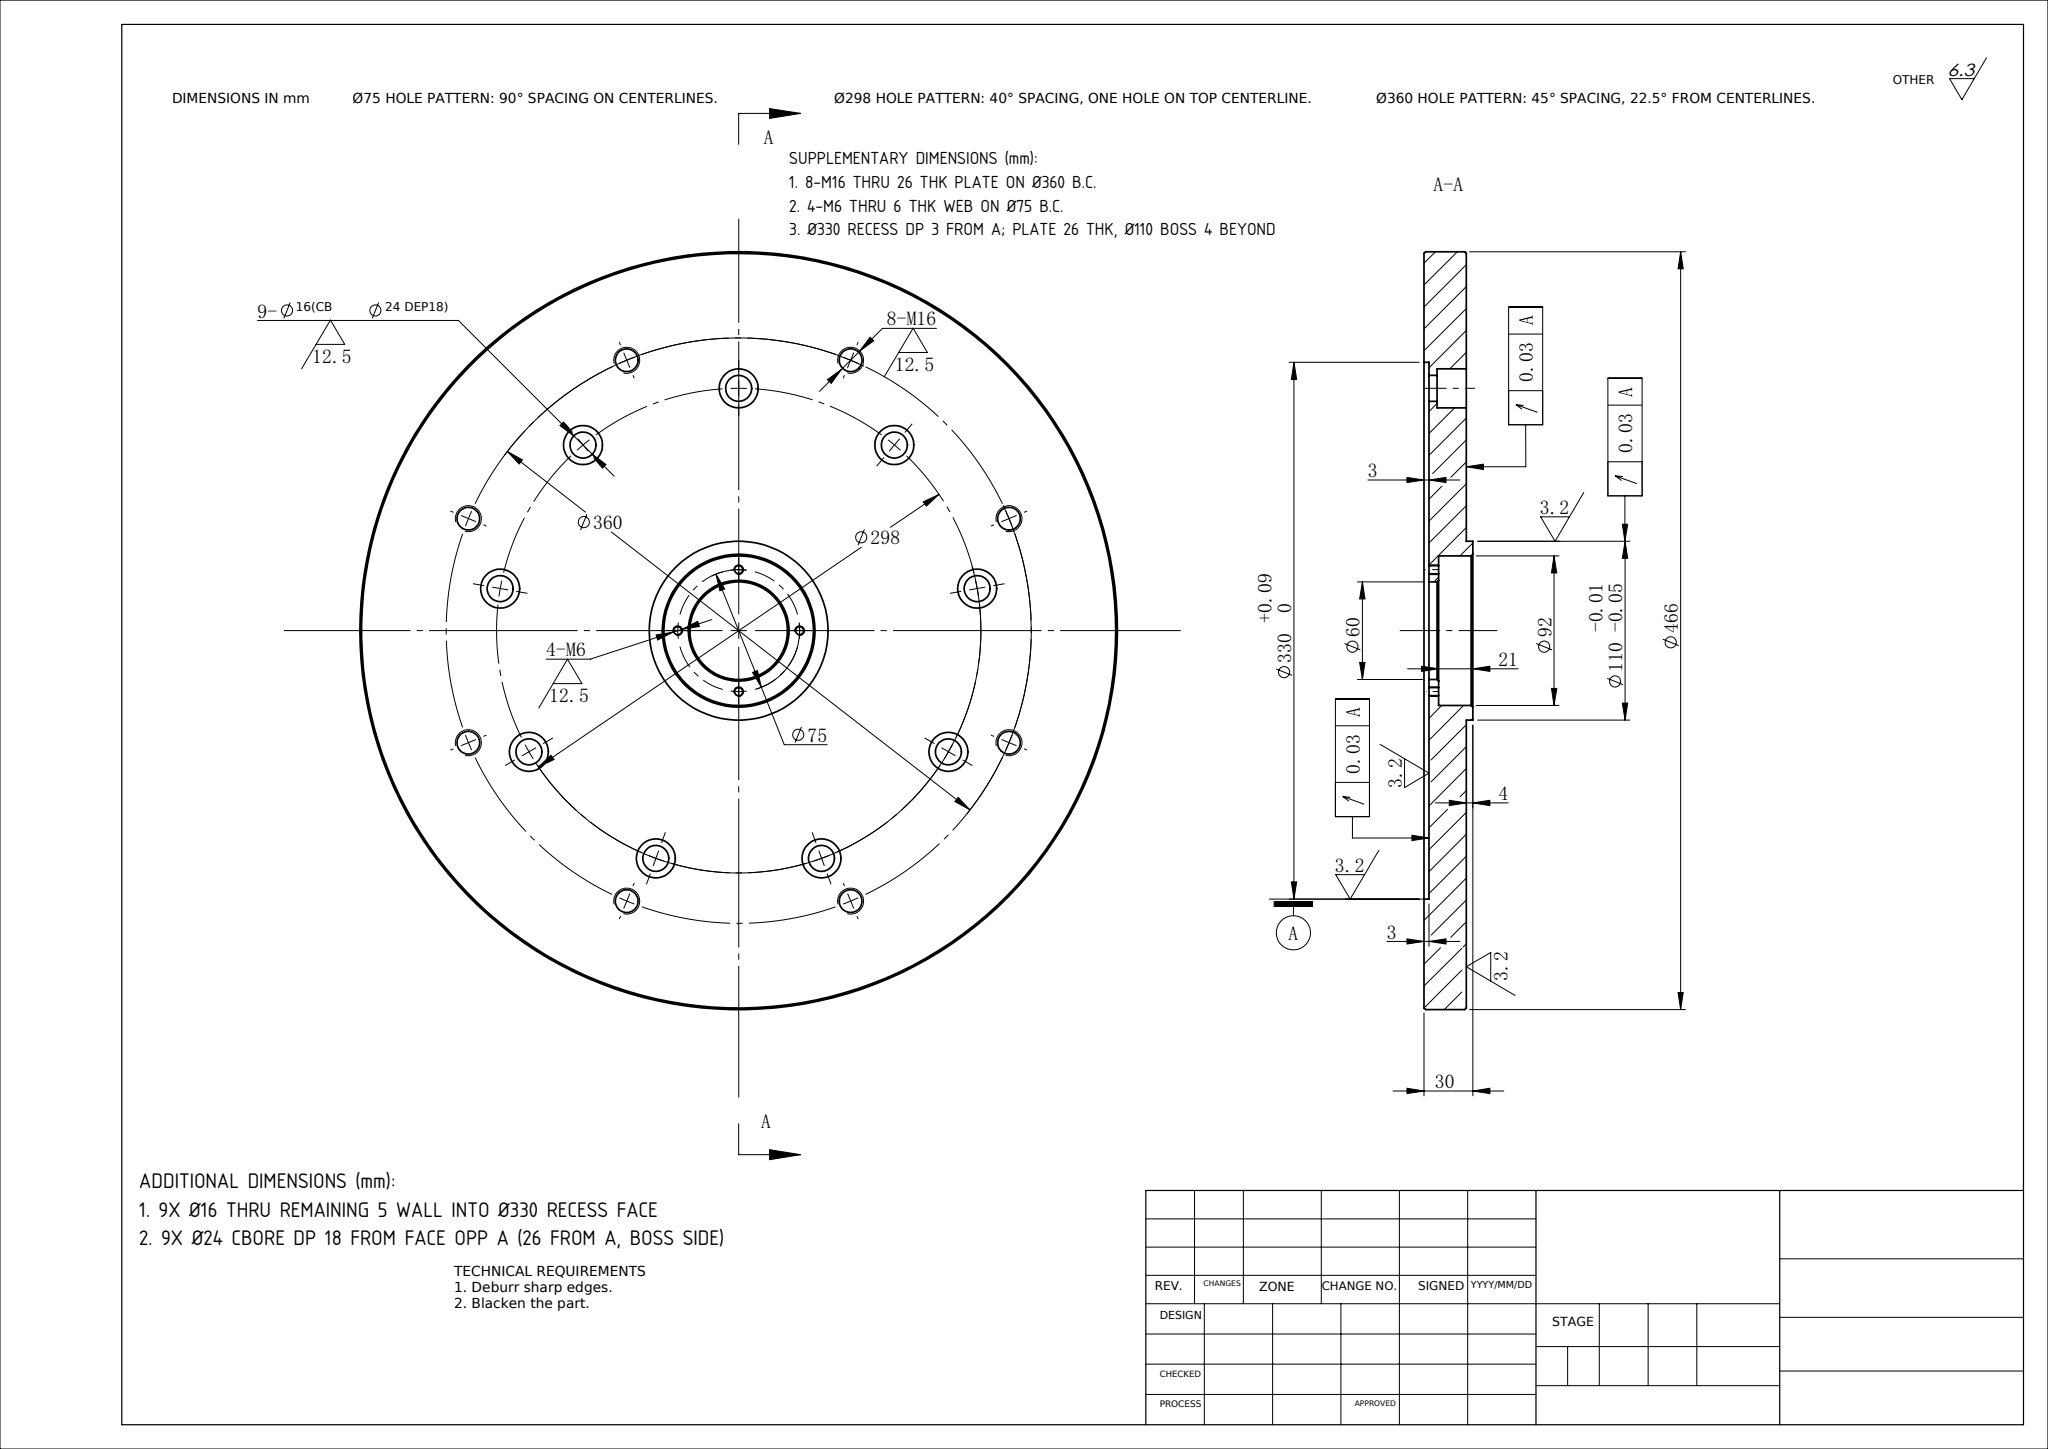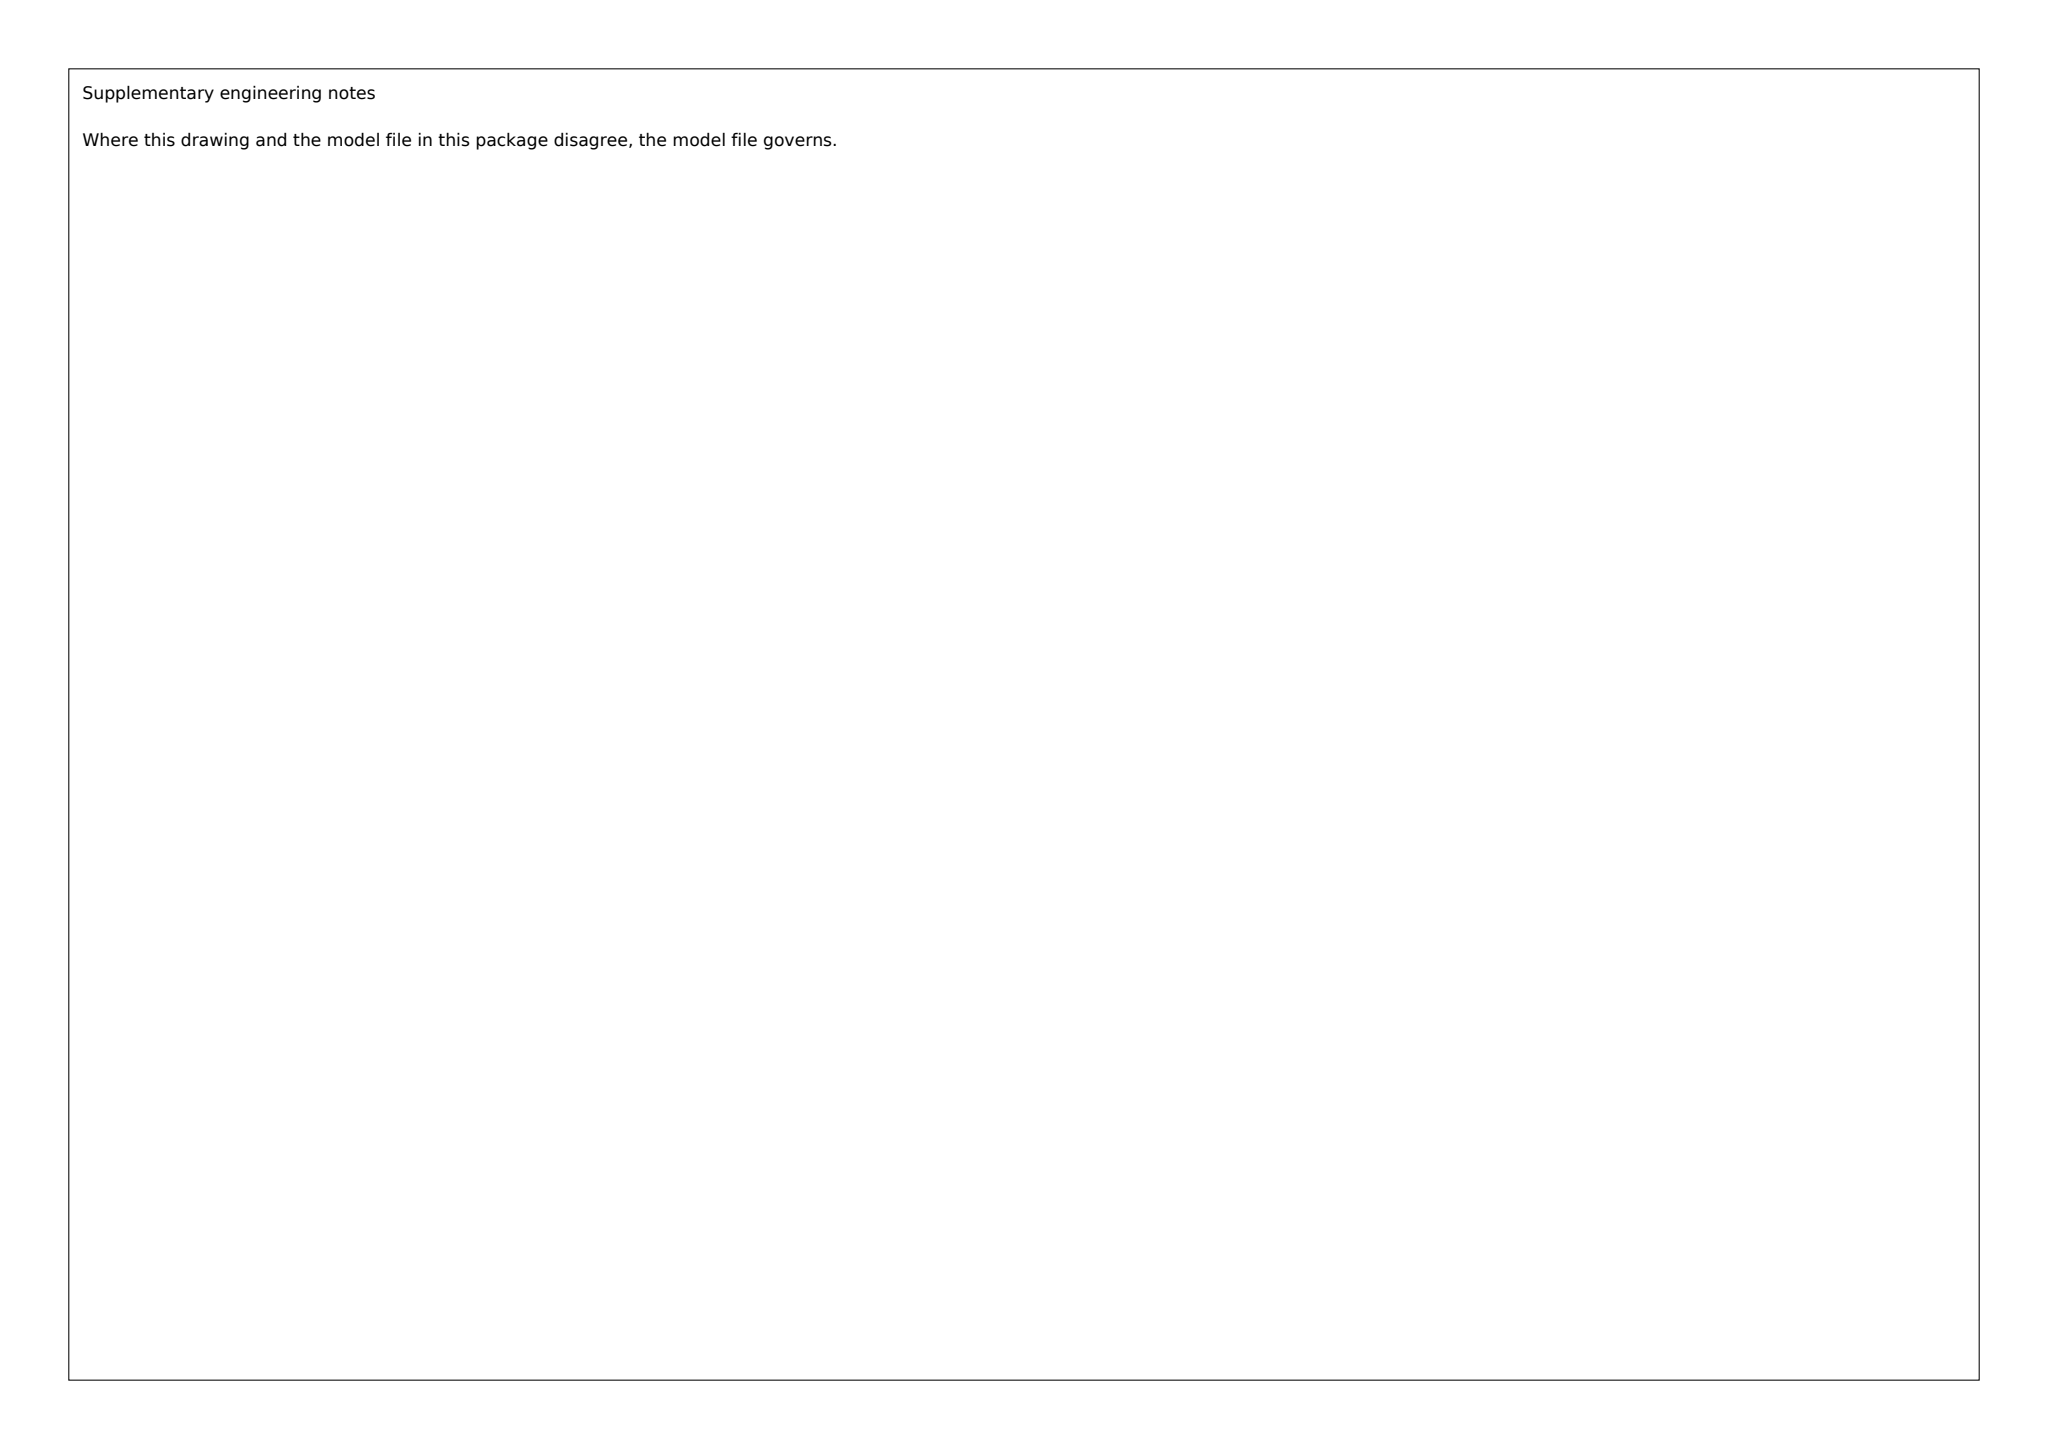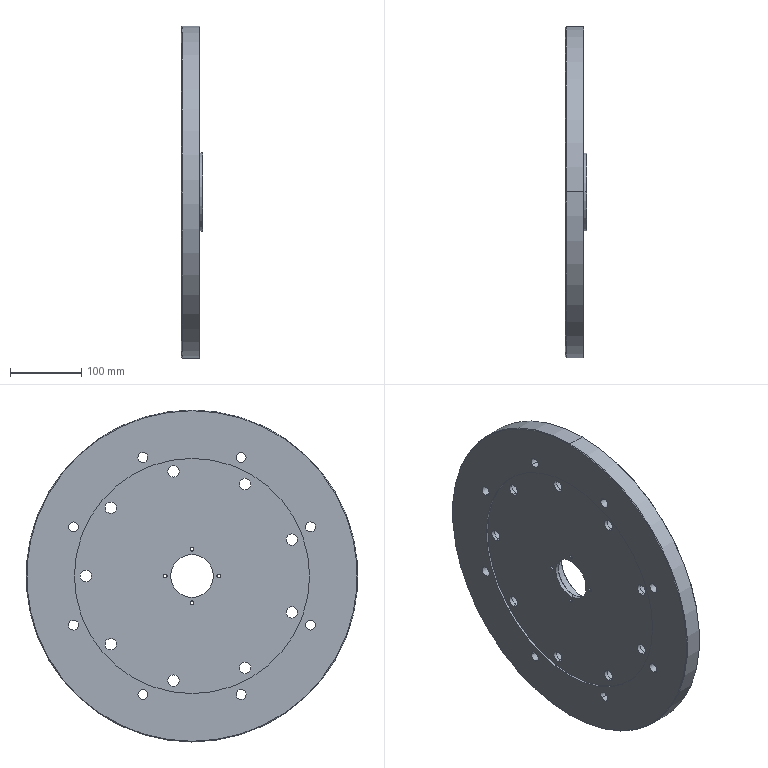Part | SolidWorks | mm | 1 solid | 92 faces | box 30 x 466 x 466 mm | volume 3942733 mm3 | cylinder 70 | plane 14 | cone 8 | commonest cylinder face diameters 24 x18 16 x18 14 x16 5 x8 110 x2 330 x2 92 x2 60 x2
build123d program:
from build123d import *

# Parameters (mm, degrees)
SKETCH10_OUTSIDE_W                                   = 599.942
SKETCH10_OUTSIDE_H                                   = 599.942
SKETCH10_OUTSIDE_R                                   = 55
CUT_EXTRUDE8_DEPTH                                   = 4
CHAMFER1_SIZE                                        = 1
HOLE_SIZE_ACCORDING_TO_HEXALOBULAR_SOCKE_D           = 16
HOLE_SIZE_ACCORDING_TO_HEXALOBULAR_SOCKE_CBORE_D     = 24
HOLE_SIZE_ACCORDING_TO_HEXALOBULAR_SOCKE_CBORE_DEPTH = 18
CIRPATTERN1_COUNT                                    = 9
M6_TAPPED_HOLE1_D                                    = 5
CIRPATTERN2_COUNT                                    = 4
M16_TAPPED_HOLE1_D                                   = 14
CIRPATTERN4_COUNT                                    = 8


with BuildPart() as part:
    # Sketch1 → Revolve1 (revolve)
    with BuildSketch(Plane.XY, mode=Mode.PRIVATE) as revolve1_sk:
        Polygon((0, 30), (6, 30), (6, 46), (27, 46), (27, 233), (-3, 233), (-3, 165), (0, 165), align=None)
    revolve(revolve1_sk.sketch.rotate(Axis((0, 0, 0), (1, 0, 0)), 90), axis=Axis((0, 0, 0), (1, 0, 0)))

    # Sketch10 outside → Cut-Extrude8 (cut)
    with BuildSketch(Plane(origin=(27, 0, 0), x_dir=(0, 0, -1), z_dir=(1, 0, 0))):
        Rectangle(SKETCH10_OUTSIDE_W, SKETCH10_OUTSIDE_H)
        Circle(SKETCH10_OUTSIDE_R, mode=Mode.SUBTRACT)
    extrude(amount=-CUT_EXTRUDE8_DEPTH, mode=Mode.SUBTRACT)

    # Chamfer1
    chamfer1_edges = [part.edges().sort_by_distance(p)[0] for p in [
        (23, 0, -233),
        (-3, 0, -233),
        (27, 0, -46),
        (6, 0, -30),
    ]]
    chamfer(chamfer1_edges, length=CHAMFER1_SIZE)

    # Hole Size according to Hexalobular Socke (through all)
    with Locations(Plane(origin=(23, -6.222, 92.291), x_dir=(0, 0, -1), z_dir=(1, 0, 0))):
        with Locations((92.291, 155.222)):
            hole_size_according_to_hexalobular_socke = CounterBoreHole(HOLE_SIZE_ACCORDING_TO_HEXALOBULAR_SOCKE_D / 2, HOLE_SIZE_ACCORDING_TO_HEXALOBULAR_SOCKE_CBORE_D / 2, HOLE_SIZE_ACCORDING_TO_HEXALOBULAR_SOCKE_CBORE_DEPTH)

    # CirPattern1: Hole Size according to Hexalobular Socke ×9 about axis
    cirpattern1_axis = Axis((0, 0, 0), (1, 0, 0))
    for i in range(1, CIRPATTERN1_COUNT):
        add(hole_size_according_to_hexalobular_socke.rotate(cirpattern1_axis, i * 360 / CIRPATTERN1_COUNT), mode=Mode.SUBTRACT)

    # M6 Tapped Hole1 (through all)
    with Locations(Plane(origin=(6, 0, 0), x_dir=(0, 0, -1), z_dir=(1, 0, 0))):
        with Locations((0, 37.5)):
            m6_tapped_hole1 = Hole(M6_TAPPED_HOLE1_D / 2)

    # CirPattern2: M6 Tapped Hole1 ×4 about axis
    cirpattern2_axis = Axis((0, 0, 0), (1, 0, 0))
    for i in range(1, CIRPATTERN2_COUNT):
        add(m6_tapped_hole1.rotate(cirpattern2_axis, i * 360 / CIRPATTERN2_COUNT), mode=Mode.SUBTRACT)

    # M16 Tapped Hole1 (through all)
    with Locations(Plane(origin=(27, 57.326, 31.838), x_dir=(0, 0, -1), z_dir=(1, 0, 0))):
        with Locations((-37.045, 108.972)):
            m16_tapped_hole1 = Hole(M16_TAPPED_HOLE1_D / 2)

    # CirPattern4: M16 Tapped Hole1 ×8 about axis
    cirpattern4_axis = Axis((0, 0, 0), (1, 0, 0))
    for i in range(1, CIRPATTERN4_COUNT):
        add(m16_tapped_hole1.rotate(cirpattern4_axis, i * 360 / CIRPATTERN4_COUNT), mode=Mode.SUBTRACT)


solid = part.part